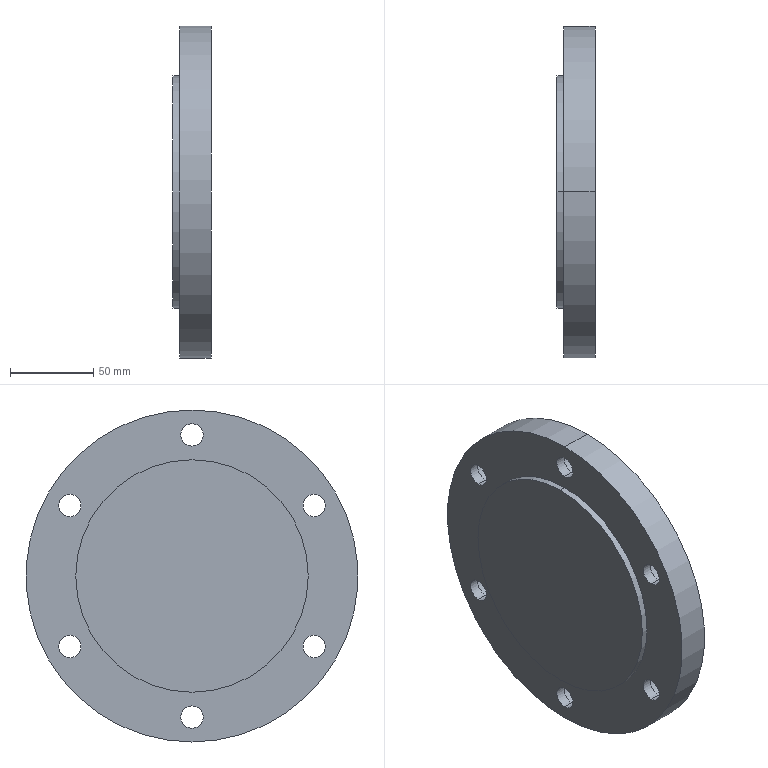Component | SolidWorks | JF21-80.1-30-1-SOLID1-1 | 1 solid | 37 faces | box 23 x 200 x 200 mm | volume 623674 mm3 | cylinder 28 | plane 9 | commonest cylinder face diameters 13.5 x12 22 x12 140 x2 200 x2
STEP:
#1=CARTESIAN_POINT('',(17.244,2.898,23.022));
#2=VERTEX_POINT('',#1);
#3=CARTESIAN_POINT('',(17.244,2.898,23.553));
#4=VERTEX_POINT('',#3);
#5=CARTESIAN_POINT('',(17.244,2.898,23.287));
#6=DIRECTION('',(-1.,0.,0.));
#7=DIRECTION('',(0.,0.,1.));
#8=AXIS2_PLACEMENT_3D('',#5,#6,#7);
#9=CIRCLE('',#8,0.2657);
#10=EDGE_CURVE('',#2,#4,#9,.T.);
#11=ORIENTED_EDGE('',*,*,#10,.T.);
#12=CARTESIAN_POINT('',(17.48,2.898,23.553));
#13=VERTEX_POINT('',#12);
#14=CARTESIAN_POINT('',(17.992,2.898,23.553));
#15=DIRECTION('',(-1.,0.,0.));
#16=VECTOR('',#15,39.37);
#17=LINE('',#14,#16);
#18=EDGE_CURVE('',#13,#4,#17,.T.);
#19=ORIENTED_EDGE('',*,*,#18,.F.);
#20=CARTESIAN_POINT('',(17.48,2.898,23.022));
#21=VERTEX_POINT('',#20);
#22=CARTESIAN_POINT('',(17.48,2.898,23.287));
#23=DIRECTION('',(1.,0.,0.));
#24=DIRECTION('',(0.,0.,-1.));
#25=AXIS2_PLACEMENT_3D('',#22,#23,#24);
#26=CIRCLE('',#25,0.2657);
#27=EDGE_CURVE('',#13,#21,#26,.T.);
#28=ORIENTED_EDGE('',*,*,#27,.T.);
#29=CARTESIAN_POINT('',(17.992,2.898,23.022));
#30=DIRECTION('',(-1.,0.,0.));
#31=VECTOR('',#30,39.37);
#32=LINE('',#29,#31);
#33=EDGE_CURVE('',#21,#2,#32,.T.);
#34=ORIENTED_EDGE('',*,*,#33,.T.);
#35=EDGE_LOOP('',(#11,#19,#28,#34));
#36=FACE_OUTER_BOUND('',#35,.T.);
#37=CARTESIAN_POINT('',(17.992,2.898,23.287));
#38=DIRECTION('',(1.,0.,0.));
#39=DIRECTION('',(0.,0.,1.));
#40=AXIS2_PLACEMENT_3D('',#37,#38,#39);
#41=CYLINDRICAL_SURFACE('',#40,0.2657);
#42=ADVANCED_FACE('',(#36),#41,.F.);
#43=CARTESIAN_POINT('',(17.48,2.898,23.72));
#44=VERTEX_POINT('',#43);
#45=CARTESIAN_POINT('',(17.48,2.898,22.854));
#46=VERTEX_POINT('',#45);
#47=CARTESIAN_POINT('',(17.48,2.898,23.287));
#48=DIRECTION('',(1.,0.,0.));
#49=DIRECTION('',(0.,0.,-1.));
#50=AXIS2_PLACEMENT_3D('',#47,#48,#49);
#51=CIRCLE('',#50,0.4331);
#52=EDGE_CURVE('',#44,#46,#51,.T.);
#53=ORIENTED_EDGE('',*,*,#52,.F.);
#54=CARTESIAN_POINT('',(17.992,2.898,23.72));
#55=VERTEX_POINT('',#54);
#56=CARTESIAN_POINT('',(17.992,2.898,23.72));
#57=DIRECTION('',(-1.,0.,0.));
#58=VECTOR('',#57,39.37);
#59=LINE('',#56,#58);
#60=EDGE_CURVE('',#55,#44,#59,.T.);
#61=ORIENTED_EDGE('',*,*,#60,.F.);
#62=CARTESIAN_POINT('',(17.992,2.898,22.854));
#63=VERTEX_POINT('',#62);
#64=CARTESIAN_POINT('',(17.992,2.898,23.287));
#65=DIRECTION('',(1.,0.,0.));
#66=DIRECTION('',(0.,0.,-1.));
#67=AXIS2_PLACEMENT_3D('',#64,#65,#66);
#68=CIRCLE('',#67,0.4331);
#69=EDGE_CURVE('',#55,#63,#68,.T.);
#70=ORIENTED_EDGE('',*,*,#69,.T.);
#71=CARTESIAN_POINT('',(17.992,2.898,22.854));
#72=DIRECTION('',(-1.,0.,0.));
#73=VECTOR('',#72,39.37);
#74=LINE('',#71,#73);
#75=EDGE_CURVE('',#63,#46,#74,.T.);
#76=ORIENTED_EDGE('',*,*,#75,.T.);
#77=EDGE_LOOP('',(#53,#61,#70,#76));
#78=FACE_OUTER_BOUND('',#77,.T.);
#79=CARTESIAN_POINT('',(17.992,2.898,23.287));
#80=DIRECTION('',(1.,0.,0.));
#81=DIRECTION('',(0.,0.,1.));
#82=AXIS2_PLACEMENT_3D('',#79,#80,#81);
#83=CYLINDRICAL_SURFACE('',#82,0.4331);
#84=ADVANCED_FACE('',(#78),#83,.F.);
#85=CARTESIAN_POINT('',(17.244,2.898,19.675));
#86=VERTEX_POINT('',#85);
#87=CARTESIAN_POINT('',(17.244,2.898,20.207));
#88=VERTEX_POINT('',#87);
#89=CARTESIAN_POINT('',(17.244,2.898,19.941));
#90=DIRECTION('',(-1.,0.,0.));
#91=DIRECTION('',(0.,0.,1.));
#92=AXIS2_PLACEMENT_3D('',#89,#90,#91);
#93=CIRCLE('',#92,0.2657);
#94=EDGE_CURVE('',#86,#88,#93,.T.);
#95=ORIENTED_EDGE('',*,*,#94,.T.);
#96=CARTESIAN_POINT('',(17.48,2.898,20.207));
#97=VERTEX_POINT('',#96);
#98=CARTESIAN_POINT('',(17.992,2.898,20.207));
#99=DIRECTION('',(-1.,0.,0.));
#100=VECTOR('',#99,39.37);
#101=LINE('',#98,#100);
#102=EDGE_CURVE('',#97,#88,#101,.T.);
#103=ORIENTED_EDGE('',*,*,#102,.F.);
#104=CARTESIAN_POINT('',(17.48,2.898,19.675));
#105=VERTEX_POINT('',#104);
#106=CARTESIAN_POINT('',(17.48,2.898,19.941));
#107=DIRECTION('',(1.,0.,0.));
#108=DIRECTION('',(0.,0.,-1.));
#109=AXIS2_PLACEMENT_3D('',#106,#107,#108);
#110=CIRCLE('',#109,0.2657);
#111=EDGE_CURVE('',#97,#105,#110,.T.);
#112=ORIENTED_EDGE('',*,*,#111,.T.);
#113=CARTESIAN_POINT('',(17.992,2.898,19.675));
#114=DIRECTION('',(-1.,0.,0.));
#115=VECTOR('',#114,39.37);
#116=LINE('',#113,#115);
#117=EDGE_CURVE('',#105,#86,#116,.T.);
#118=ORIENTED_EDGE('',*,*,#117,.T.);
#119=EDGE_LOOP('',(#95,#103,#112,#118));
#120=FACE_OUTER_BOUND('',#119,.T.);
#121=CARTESIAN_POINT('',(17.992,2.898,19.941));
#122=DIRECTION('',(1.,0.,0.));
#123=DIRECTION('',(0.,0.,1.));
#124=AXIS2_PLACEMENT_3D('',#121,#122,#123);
#125=CYLINDRICAL_SURFACE('',#124,0.2657);
#126=ADVANCED_FACE('',(#120),#125,.F.);
#127=CARTESIAN_POINT('',(17.48,2.898,20.374));
#128=VERTEX_POINT('',#127);
#129=CARTESIAN_POINT('',(17.48,2.898,19.508));
#130=VERTEX_POINT('',#129);
#131=CARTESIAN_POINT('',(17.48,2.898,19.941));
#132=DIRECTION('',(1.,0.,0.));
#133=DIRECTION('',(0.,0.,-1.));
#134=AXIS2_PLACEMENT_3D('',#131,#132,#133);
#135=CIRCLE('',#134,0.4331);
#136=EDGE_CURVE('',#128,#130,#135,.T.);
#137=ORIENTED_EDGE('',*,*,#136,.F.);
#138=CARTESIAN_POINT('',(17.992,2.898,20.374));
#139=VERTEX_POINT('',#138);
#140=CARTESIAN_POINT('',(17.992,2.898,20.374));
#141=DIRECTION('',(-1.,0.,0.));
#142=VECTOR('',#141,39.37);
#143=LINE('',#140,#142);
#144=EDGE_CURVE('',#139,#128,#143,.T.);
#145=ORIENTED_EDGE('',*,*,#144,.F.);
#146=CARTESIAN_POINT('',(17.992,2.898,19.508));
#147=VERTEX_POINT('',#146);
#148=CARTESIAN_POINT('',(17.992,2.898,19.941));
#149=DIRECTION('',(1.,0.,0.));
#150=DIRECTION('',(0.,0.,-1.));
#151=AXIS2_PLACEMENT_3D('',#148,#149,#150);
#152=CIRCLE('',#151,0.4331);
#153=EDGE_CURVE('',#139,#147,#152,.T.);
#154=ORIENTED_EDGE('',*,*,#153,.T.);
#155=CARTESIAN_POINT('',(17.992,2.898,19.508));
#156=DIRECTION('',(-1.,0.,0.));
#157=VECTOR('',#156,39.37);
#158=LINE('',#155,#157);
#159=EDGE_CURVE('',#147,#130,#158,.T.);
#160=ORIENTED_EDGE('',*,*,#159,.T.);
#161=EDGE_LOOP('',(#137,#145,#154,#160));
#162=FACE_OUTER_BOUND('',#161,.T.);
#163=CARTESIAN_POINT('',(17.992,2.898,19.941));
#164=DIRECTION('',(1.,0.,0.));
#165=DIRECTION('',(0.,0.,1.));
#166=AXIS2_PLACEMENT_3D('',#163,#164,#165);
#167=CYLINDRICAL_SURFACE('',#166,0.4331);
#168=ADVANCED_FACE('',(#162),#167,.F.);
#169=CARTESIAN_POINT('',(17.244,-0.,18.002));
#170=VERTEX_POINT('',#169);
#171=CARTESIAN_POINT('',(17.244,-0.,18.533));
#172=VERTEX_POINT('',#171);
#173=CARTESIAN_POINT('',(17.244,-0.,18.268));
#174=DIRECTION('',(-1.,0.,0.));
#175=DIRECTION('',(0.,0.,1.));
#176=AXIS2_PLACEMENT_3D('',#173,#174,#175);
#177=CIRCLE('',#176,0.2657);
#178=EDGE_CURVE('',#170,#172,#177,.T.);
#179=ORIENTED_EDGE('',*,*,#178,.T.);
#180=CARTESIAN_POINT('',(17.48,-0.,18.533));
#181=VERTEX_POINT('',#180);
#182=CARTESIAN_POINT('',(17.992,-0.,18.533));
#183=DIRECTION('',(-1.,0.,0.));
#184=VECTOR('',#183,39.37);
#185=LINE('',#182,#184);
#186=EDGE_CURVE('',#181,#172,#185,.T.);
#187=ORIENTED_EDGE('',*,*,#186,.F.);
#188=CARTESIAN_POINT('',(17.48,-0.,18.002));
#189=VERTEX_POINT('',#188);
#190=CARTESIAN_POINT('',(17.48,-0.,18.268));
#191=DIRECTION('',(1.,0.,0.));
#192=DIRECTION('',(0.,0.,-1.));
#193=AXIS2_PLACEMENT_3D('',#190,#191,#192);
#194=CIRCLE('',#193,0.2657);
#195=EDGE_CURVE('',#181,#189,#194,.T.);
#196=ORIENTED_EDGE('',*,*,#195,.T.);
#197=CARTESIAN_POINT('',(17.992,-0.,18.002));
#198=DIRECTION('',(-1.,0.,0.));
#199=VECTOR('',#198,39.37);
#200=LINE('',#197,#199);
#201=EDGE_CURVE('',#189,#170,#200,.T.);
#202=ORIENTED_EDGE('',*,*,#201,.T.);
#203=EDGE_LOOP('',(#179,#187,#196,#202));
#204=FACE_OUTER_BOUND('',#203,.T.);
#205=CARTESIAN_POINT('',(17.992,-0.,18.268));
#206=DIRECTION('',(1.,0.,0.));
#207=DIRECTION('',(0.,0.,1.));
#208=AXIS2_PLACEMENT_3D('',#205,#206,#207);
#209=CYLINDRICAL_SURFACE('',#208,0.2657);
#210=ADVANCED_FACE('',(#204),#209,.F.);
#211=CARTESIAN_POINT('',(17.48,-0.,18.701));
#212=VERTEX_POINT('',#211);
#213=CARTESIAN_POINT('',(17.48,-0.,17.835));
#214=VERTEX_POINT('',#213);
#215=CARTESIAN_POINT('',(17.48,-0.,18.268));
#216=DIRECTION('',(1.,0.,0.));
#217=DIRECTION('',(0.,0.,-1.));
#218=AXIS2_PLACEMENT_3D('',#215,#216,#217);
#219=CIRCLE('',#218,0.4331);
#220=EDGE_CURVE('',#212,#214,#219,.T.);
#221=ORIENTED_EDGE('',*,*,#220,.F.);
#222=CARTESIAN_POINT('',(17.992,-0.,18.701));
#223=VERTEX_POINT('',#222);
#224=CARTESIAN_POINT('',(17.992,-0.,18.701));
#225=DIRECTION('',(-1.,0.,0.));
#226=VECTOR('',#225,39.37);
#227=LINE('',#224,#226);
#228=EDGE_CURVE('',#223,#212,#227,.T.);
#229=ORIENTED_EDGE('',*,*,#228,.F.);
#230=CARTESIAN_POINT('',(17.992,-0.,17.835));
#231=VERTEX_POINT('',#230);
#232=CARTESIAN_POINT('',(17.992,-0.,18.268));
#233=DIRECTION('',(1.,0.,0.));
#234=DIRECTION('',(0.,0.,-1.));
#235=AXIS2_PLACEMENT_3D('',#232,#233,#234);
#236=CIRCLE('',#235,0.4331);
#237=EDGE_CURVE('',#223,#231,#236,.T.);
#238=ORIENTED_EDGE('',*,*,#237,.T.);
#239=CARTESIAN_POINT('',(17.992,-0.,17.835));
#240=DIRECTION('',(-1.,0.,0.));
#241=VECTOR('',#240,39.37);
#242=LINE('',#239,#241);
#243=EDGE_CURVE('',#231,#214,#242,.T.);
#244=ORIENTED_EDGE('',*,*,#243,.T.);
#245=EDGE_LOOP('',(#221,#229,#238,#244));
#246=FACE_OUTER_BOUND('',#245,.T.);
#247=CARTESIAN_POINT('',(17.992,-0.,18.268));
#248=DIRECTION('',(1.,0.,0.));
#249=DIRECTION('',(0.,0.,1.));
#250=AXIS2_PLACEMENT_3D('',#247,#248,#249);
#251=CYLINDRICAL_SURFACE('',#250,0.4331);
#252=ADVANCED_FACE('',(#246),#251,.F.);
#253=CARTESIAN_POINT('',(17.244,-2.898,19.675));
#254=VERTEX_POINT('',#253);
#255=CARTESIAN_POINT('',(17.244,-2.898,20.207));
#256=VERTEX_POINT('',#255);
#257=CARTESIAN_POINT('',(17.244,-2.898,19.941));
#258=DIRECTION('',(-1.,0.,0.));
#259=DIRECTION('',(0.,0.,1.));
#260=AXIS2_PLACEMENT_3D('',#257,#258,#259);
#261=CIRCLE('',#260,0.2657);
#262=EDGE_CURVE('',#254,#256,#261,.T.);
#263=ORIENTED_EDGE('',*,*,#262,.T.);
#264=CARTESIAN_POINT('',(17.48,-2.898,20.207));
#265=VERTEX_POINT('',#264);
#266=CARTESIAN_POINT('',(17.992,-2.898,20.207));
#267=DIRECTION('',(-1.,0.,0.));
#268=VECTOR('',#267,39.37);
#269=LINE('',#266,#268);
#270=EDGE_CURVE('',#265,#256,#269,.T.);
#271=ORIENTED_EDGE('',*,*,#270,.F.);
#272=CARTESIAN_POINT('',(17.48,-2.898,19.675));
#273=VERTEX_POINT('',#272);
#274=CARTESIAN_POINT('',(17.48,-2.898,19.941));
#275=DIRECTION('',(1.,0.,0.));
#276=DIRECTION('',(0.,0.,-1.));
#277=AXIS2_PLACEMENT_3D('',#274,#275,#276);
#278=CIRCLE('',#277,0.2657);
#279=EDGE_CURVE('',#265,#273,#278,.T.);
#280=ORIENTED_EDGE('',*,*,#279,.T.);
#281=CARTESIAN_POINT('',(17.992,-2.898,19.675));
#282=DIRECTION('',(-1.,0.,0.));
#283=VECTOR('',#282,39.37);
#284=LINE('',#281,#283);
#285=EDGE_CURVE('',#273,#254,#284,.T.);
#286=ORIENTED_EDGE('',*,*,#285,.T.);
#287=EDGE_LOOP('',(#263,#271,#280,#286));
#288=FACE_OUTER_BOUND('',#287,.T.);
#289=CARTESIAN_POINT('',(17.992,-2.898,19.941));
#290=DIRECTION('',(1.,0.,0.));
#291=DIRECTION('',(0.,0.,1.));
#292=AXIS2_PLACEMENT_3D('',#289,#290,#291);
#293=CYLINDRICAL_SURFACE('',#292,0.2657);
#294=ADVANCED_FACE('',(#288),#293,.F.);
#295=CARTESIAN_POINT('',(17.48,-2.898,20.374));
#296=VERTEX_POINT('',#295);
#297=CARTESIAN_POINT('',(17.48,-2.898,19.508));
#298=VERTEX_POINT('',#297);
#299=CARTESIAN_POINT('',(17.48,-2.898,19.941));
#300=DIRECTION('',(1.,0.,0.));
#301=DIRECTION('',(0.,0.,-1.));
#302=AXIS2_PLACEMENT_3D('',#299,#300,#301);
#303=CIRCLE('',#302,0.4331);
#304=EDGE_CURVE('',#296,#298,#303,.T.);
#305=ORIENTED_EDGE('',*,*,#304,.F.);
#306=CARTESIAN_POINT('',(17.992,-2.898,20.374));
#307=VERTEX_POINT('',#306);
#308=CARTESIAN_POINT('',(17.992,-2.898,20.374));
#309=DIRECTION('',(-1.,0.,0.));
#310=VECTOR('',#309,39.37);
#311=LINE('',#308,#310);
#312=EDGE_CURVE('',#307,#296,#311,.T.);
#313=ORIENTED_EDGE('',*,*,#312,.F.);
#314=CARTESIAN_POINT('',(17.992,-2.898,19.508));
#315=VERTEX_POINT('',#314);
#316=CARTESIAN_POINT('',(17.992,-2.898,19.941));
#317=DIRECTION('',(1.,0.,0.));
#318=DIRECTION('',(0.,0.,-1.));
#319=AXIS2_PLACEMENT_3D('',#316,#317,#318);
#320=CIRCLE('',#319,0.4331);
#321=EDGE_CURVE('',#307,#315,#320,.T.);
#322=ORIENTED_EDGE('',*,*,#321,.T.);
#323=CARTESIAN_POINT('',(17.992,-2.898,19.508));
#324=DIRECTION('',(-1.,0.,0.));
#325=VECTOR('',#324,39.37);
#326=LINE('',#323,#325);
#327=EDGE_CURVE('',#315,#298,#326,.T.);
#328=ORIENTED_EDGE('',*,*,#327,.T.);
#329=EDGE_LOOP('',(#305,#313,#322,#328));
#330=FACE_OUTER_BOUND('',#329,.T.);
#331=CARTESIAN_POINT('',(17.992,-2.898,19.941));
#332=DIRECTION('',(1.,0.,0.));
#333=DIRECTION('',(0.,0.,1.));
#334=AXIS2_PLACEMENT_3D('',#331,#332,#333);
#335=CYLINDRICAL_SURFACE('',#334,0.4331);
#336=ADVANCED_FACE('',(#330),#335,.F.);
#337=CARTESIAN_POINT('',(17.244,-2.898,23.022));
#338=VERTEX_POINT('',#337);
#339=CARTESIAN_POINT('',(17.244,-2.898,23.553));
#340=VERTEX_POINT('',#339);
#341=CARTESIAN_POINT('',(17.244,-2.898,23.287));
#342=DIRECTION('',(-1.,0.,0.));
#343=DIRECTION('',(0.,0.,1.));
#344=AXIS2_PLACEMENT_3D('',#341,#342,#343);
#345=CIRCLE('',#344,0.2657);
#346=EDGE_CURVE('',#338,#340,#345,.T.);
#347=ORIENTED_EDGE('',*,*,#346,.T.);
#348=CARTESIAN_POINT('',(17.48,-2.898,23.553));
#349=VERTEX_POINT('',#348);
#350=CARTESIAN_POINT('',(17.992,-2.898,23.553));
#351=DIRECTION('',(-1.,0.,0.));
#352=VECTOR('',#351,39.37);
#353=LINE('',#350,#352);
#354=EDGE_CURVE('',#349,#340,#353,.T.);
#355=ORIENTED_EDGE('',*,*,#354,.F.);
#356=CARTESIAN_POINT('',(17.48,-2.898,23.022));
#357=VERTEX_POINT('',#356);
#358=CARTESIAN_POINT('',(17.48,-2.898,23.287));
#359=DIRECTION('',(1.,0.,0.));
#360=DIRECTION('',(0.,0.,-1.));
#361=AXIS2_PLACEMENT_3D('',#358,#359,#360);
#362=CIRCLE('',#361,0.2657);
#363=EDGE_CURVE('',#349,#357,#362,.T.);
#364=ORIENTED_EDGE('',*,*,#363,.T.);
#365=CARTESIAN_POINT('',(17.992,-2.898,23.022));
#366=DIRECTION('',(-1.,0.,0.));
#367=VECTOR('',#366,39.37);
#368=LINE('',#365,#367);
#369=EDGE_CURVE('',#357,#338,#368,.T.);
#370=ORIENTED_EDGE('',*,*,#369,.T.);
#371=EDGE_LOOP('',(#347,#355,#364,#370));
#372=FACE_OUTER_BOUND('',#371,.T.);
#373=CARTESIAN_POINT('',(17.992,-2.898,23.287));
#374=DIRECTION('',(1.,0.,0.));
#375=DIRECTION('',(0.,0.,1.));
#376=AXIS2_PLACEMENT_3D('',#373,#374,#375);
#377=CYLINDRICAL_SURFACE('',#376,0.2657);
#378=ADVANCED_FACE('',(#372),#377,.F.);
#379=CARTESIAN_POINT('',(17.48,-2.898,23.72));
#380=VERTEX_POINT('',#379);
#381=CARTESIAN_POINT('',(17.48,-2.898,22.854));
#382=VERTEX_POINT('',#381);
#383=CARTESIAN_POINT('',(17.48,-2.898,23.287));
#384=DIRECTION('',(1.,0.,0.));
#385=DIRECTION('',(0.,0.,-1.));
#386=AXIS2_PLACEMENT_3D('',#383,#384,#385);
#387=CIRCLE('',#386,0.4331);
#388=EDGE_CURVE('',#380,#382,#387,.T.);
#389=ORIENTED_EDGE('',*,*,#388,.F.);
#390=CARTESIAN_POINT('',(17.992,-2.898,23.72));
#391=VERTEX_POINT('',#390);
#392=CARTESIAN_POINT('',(17.992,-2.898,23.72));
#393=DIRECTION('',(-1.,0.,0.));
#394=VECTOR('',#393,39.37);
#395=LINE('',#392,#394);
#396=EDGE_CURVE('',#391,#380,#395,.T.);
#397=ORIENTED_EDGE('',*,*,#396,.F.);
#398=CARTESIAN_POINT('',(17.992,-2.898,22.854));
#399=VERTEX_POINT('',#398);
#400=CARTESIAN_POINT('',(17.992,-2.898,23.287));
#401=DIRECTION('',(1.,0.,0.));
#402=DIRECTION('',(0.,0.,-1.));
#403=AXIS2_PLACEMENT_3D('',#400,#401,#402);
#404=CIRCLE('',#403,0.4331);
#405=EDGE_CURVE('',#391,#399,#404,.T.);
#406=ORIENTED_EDGE('',*,*,#405,.T.);
#407=CARTESIAN_POINT('',(17.992,-2.898,22.854));
#408=DIRECTION('',(-1.,0.,0.));
#409=VECTOR('',#408,39.37);
#410=LINE('',#407,#409);
#411=EDGE_CURVE('',#399,#382,#410,.T.);
#412=ORIENTED_EDGE('',*,*,#411,.T.);
#413=EDGE_LOOP('',(#389,#397,#406,#412));
#414=FACE_OUTER_BOUND('',#413,.T.);
#415=CARTESIAN_POINT('',(17.992,-2.898,23.287));
#416=DIRECTION('',(1.,0.,0.));
#417=DIRECTION('',(0.,0.,1.));
#418=AXIS2_PLACEMENT_3D('',#415,#416,#417);
#419=CYLINDRICAL_SURFACE('',#418,0.4331);
#420=ADVANCED_FACE('',(#414),#419,.F.);
#421=CARTESIAN_POINT('',(17.244,-0.,24.695));
#422=VERTEX_POINT('',#421);
#423=CARTESIAN_POINT('',(17.244,-0.,25.226));
#424=VERTEX_POINT('',#423);
#425=CARTESIAN_POINT('',(17.244,-0.,24.961));
#426=DIRECTION('',(-1.,0.,0.));
#427=DIRECTION('',(0.,0.,1.));
#428=AXIS2_PLACEMENT_3D('',#425,#426,#427);
#429=CIRCLE('',#428,0.2657);
#430=EDGE_CURVE('',#422,#424,#429,.T.);
#431=ORIENTED_EDGE('',*,*,#430,.T.);
#432=CARTESIAN_POINT('',(17.48,-0.,25.226));
#433=VERTEX_POINT('',#432);
#434=CARTESIAN_POINT('',(17.992,-0.,25.226));
#435=DIRECTION('',(-1.,0.,0.));
#436=VECTOR('',#435,39.37);
#437=LINE('',#434,#436);
#438=EDGE_CURVE('',#433,#424,#437,.T.);
#439=ORIENTED_EDGE('',*,*,#438,.F.);
#440=CARTESIAN_POINT('',(17.48,-0.,24.695));
#441=VERTEX_POINT('',#440);
#442=CARTESIAN_POINT('',(17.48,-0.,24.961));
#443=DIRECTION('',(1.,0.,0.));
#444=DIRECTION('',(0.,0.,-1.));
#445=AXIS2_PLACEMENT_3D('',#442,#443,#444);
#446=CIRCLE('',#445,0.2657);
#447=EDGE_CURVE('',#433,#441,#446,.T.);
#448=ORIENTED_EDGE('',*,*,#447,.T.);
#449=CARTESIAN_POINT('',(17.992,-0.,24.695));
#450=DIRECTION('',(-1.,0.,0.));
#451=VECTOR('',#450,39.37);
#452=LINE('',#449,#451);
#453=EDGE_CURVE('',#441,#422,#452,.T.);
#454=ORIENTED_EDGE('',*,*,#453,.T.);
#455=EDGE_LOOP('',(#431,#439,#448,#454));
#456=FACE_OUTER_BOUND('',#455,.T.);
#457=CARTESIAN_POINT('',(17.992,-0.,24.961));
#458=DIRECTION('',(1.,0.,0.));
#459=DIRECTION('',(0.,0.,1.));
#460=AXIS2_PLACEMENT_3D('',#457,#458,#459);
#461=CYLINDRICAL_SURFACE('',#460,0.2657);
#462=ADVANCED_FACE('',(#456),#461,.F.);
#463=CARTESIAN_POINT('',(17.48,-0.,25.394));
#464=VERTEX_POINT('',#463);
#465=CARTESIAN_POINT('',(17.48,-0.,24.528));
#466=VERTEX_POINT('',#465);
#467=CARTESIAN_POINT('',(17.48,-0.,24.961));
#468=DIRECTION('',(1.,0.,0.));
#469=DIRECTION('',(0.,0.,-1.));
#470=AXIS2_PLACEMENT_3D('',#467,#468,#469);
#471=CIRCLE('',#470,0.4331);
#472=EDGE_CURVE('',#464,#466,#471,.T.);
#473=ORIENTED_EDGE('',*,*,#472,.F.);
#474=CARTESIAN_POINT('',(17.992,-0.,25.394));
#475=VERTEX_POINT('',#474);
#476=CARTESIAN_POINT('',(17.992,-0.,25.394));
#477=DIRECTION('',(-1.,0.,0.));
#478=VECTOR('',#477,39.37);
#479=LINE('',#476,#478);
#480=EDGE_CURVE('',#475,#464,#479,.T.);
#481=ORIENTED_EDGE('',*,*,#480,.F.);
#482=CARTESIAN_POINT('',(17.992,-0.,24.528));
#483=VERTEX_POINT('',#482);
#484=CARTESIAN_POINT('',(17.992,-0.,24.961));
#485=DIRECTION('',(1.,0.,0.));
#486=DIRECTION('',(0.,0.,-1.));
#487=AXIS2_PLACEMENT_3D('',#484,#485,#486);
#488=CIRCLE('',#487,0.4331);
#489=EDGE_CURVE('',#475,#483,#488,.T.);
#490=ORIENTED_EDGE('',*,*,#489,.T.);
#491=CARTESIAN_POINT('',(17.992,-0.,24.528));
#492=DIRECTION('',(-1.,0.,0.));
#493=VECTOR('',#492,39.37);
#494=LINE('',#491,#493);
#495=EDGE_CURVE('',#483,#466,#494,.T.);
#496=ORIENTED_EDGE('',*,*,#495,.T.);
#497=EDGE_LOOP('',(#473,#481,#490,#496));
#498=FACE_OUTER_BOUND('',#497,.T.);
#499=CARTESIAN_POINT('',(17.992,-0.,24.961));
#500=DIRECTION('',(1.,0.,0.));
#501=DIRECTION('',(0.,0.,1.));
#502=AXIS2_PLACEMENT_3D('',#499,#500,#501);
#503=CYLINDRICAL_SURFACE('',#502,0.4331);
#504=ADVANCED_FACE('',(#498),#503,.F.);
#505=CARTESIAN_POINT('',(17.087,-0.,24.37));
#506=VERTEX_POINT('',#505);
#507=CARTESIAN_POINT('',(17.087,-0.,18.858));
#508=VERTEX_POINT('',#507);
#509=CARTESIAN_POINT('',(17.087,-0.,21.614));
#510=DIRECTION('',(-1.,0.,0.));
#511=DIRECTION('',(0.,0.,1.));
#512=AXIS2_PLACEMENT_3D('',#509,#510,#511);
#513=CIRCLE('',#512,2.756);
#514=EDGE_CURVE('',#506,#508,#513,.T.);
#515=ORIENTED_EDGE('',*,*,#514,.F.);
#516=CARTESIAN_POINT('',(17.244,-0.,24.37));
#517=VERTEX_POINT('',#516);
#518=CARTESIAN_POINT('',(17.087,-0.,24.37));
#519=DIRECTION('',(-1.,0.,0.));
#520=VECTOR('',#519,39.37);
#521=LINE('',#518,#520);
#522=EDGE_CURVE('',#517,#506,#521,.T.);
#523=ORIENTED_EDGE('',*,*,#522,.F.);
#524=CARTESIAN_POINT('',(17.244,-0.,18.858));
#525=VERTEX_POINT('',#524);
#526=CARTESIAN_POINT('',(17.244,-0.,21.614));
#527=DIRECTION('',(-1.,0.,0.));
#528=DIRECTION('',(0.,0.,1.));
#529=AXIS2_PLACEMENT_3D('',#526,#527,#528);
#530=CIRCLE('',#529,2.756);
#531=EDGE_CURVE('',#517,#525,#530,.T.);
#532=ORIENTED_EDGE('',*,*,#531,.T.);
#533=CARTESIAN_POINT('',(17.087,-0.,18.858));
#534=DIRECTION('',(-1.,0.,0.));
#535=VECTOR('',#534,39.37);
#536=LINE('',#533,#535);
#537=EDGE_CURVE('',#525,#508,#536,.T.);
#538=ORIENTED_EDGE('',*,*,#537,.T.);
#539=EDGE_LOOP('',(#515,#523,#532,#538));
#540=FACE_OUTER_BOUND('',#539,.T.);
#541=CARTESIAN_POINT('',(17.087,-0.,21.614));
#542=DIRECTION('',(1.,0.,0.));
#543=DIRECTION('',(0.,0.,1.));
#544=AXIS2_PLACEMENT_3D('',#541,#542,#543);
#545=CYLINDRICAL_SURFACE('',#544,2.756);
#546=ADVANCED_FACE('',(#540),#545,.T.);
#547=CARTESIAN_POINT('',(17.244,-0.,25.551));
#548=VERTEX_POINT('',#547);
#549=CARTESIAN_POINT('',(17.244,-0.,17.677));
#550=VERTEX_POINT('',#549);
#551=CARTESIAN_POINT('',(17.244,-0.,21.614));
#552=DIRECTION('',(-1.,0.,0.));
#553=DIRECTION('',(0.,0.,1.));
#554=AXIS2_PLACEMENT_3D('',#551,#552,#553);
#555=CIRCLE('',#554,3.937);
#556=EDGE_CURVE('',#548,#550,#555,.T.);
#557=ORIENTED_EDGE('',*,*,#556,.F.);
#558=CARTESIAN_POINT('',(17.992,-0.,25.551));
#559=VERTEX_POINT('',#558);
#560=CARTESIAN_POINT('',(17.244,-0.,25.551));
#561=DIRECTION('',(-1.,0.,0.));
#562=VECTOR('',#561,39.37);
#563=LINE('',#560,#562);
#564=EDGE_CURVE('',#559,#548,#563,.T.);
#565=ORIENTED_EDGE('',*,*,#564,.F.);
#566=CARTESIAN_POINT('',(17.992,-0.,17.677));
#567=VERTEX_POINT('',#566);
#568=CARTESIAN_POINT('',(17.992,-0.,21.614));
#569=DIRECTION('',(-1.,0.,0.));
#570=DIRECTION('',(0.,0.,1.));
#571=AXIS2_PLACEMENT_3D('',#568,#569,#570);
#572=CIRCLE('',#571,3.937);
#573=EDGE_CURVE('',#559,#567,#572,.T.);
#574=ORIENTED_EDGE('',*,*,#573,.T.);
#575=CARTESIAN_POINT('',(17.244,-0.,17.677));
#576=DIRECTION('',(-1.,0.,0.));
#577=VECTOR('',#576,39.37);
#578=LINE('',#575,#577);
#579=EDGE_CURVE('',#567,#550,#578,.T.);
#580=ORIENTED_EDGE('',*,*,#579,.T.);
#581=EDGE_LOOP('',(#557,#565,#574,#580));
#582=FACE_OUTER_BOUND('',#581,.T.);
#583=CARTESIAN_POINT('',(17.244,-0.,21.614));
#584=DIRECTION('',(1.,0.,0.));
#585=DIRECTION('',(0.,0.,1.));
#586=AXIS2_PLACEMENT_3D('',#583,#584,#585);
#587=CYLINDRICAL_SURFACE('',#586,3.937);
#588=ADVANCED_FACE('',(#582),#587,.T.);
#589=ORIENTED_EDGE('',*,*,#10,.F.);
#590=CARTESIAN_POINT('',(17.244,2.898,23.287));
#591=DIRECTION('',(-1.,0.,0.));
#592=DIRECTION('',(0.,0.,1.));
#593=AXIS2_PLACEMENT_3D('',#590,#591,#592);
#594=CIRCLE('',#593,0.2657);
#595=EDGE_CURVE('',#4,#2,#594,.T.);
#596=ORIENTED_EDGE('',*,*,#595,.F.);
#597=EDGE_LOOP('',(#589,#596));
#598=FACE_BOUND('',#597,.T.);
#599=ORIENTED_EDGE('',*,*,#94,.F.);
#600=CARTESIAN_POINT('',(17.244,2.898,19.941));
#601=DIRECTION('',(-1.,0.,0.));
#602=DIRECTION('',(0.,0.,1.));
#603=AXIS2_PLACEMENT_3D('',#600,#601,#602);
#604=CIRCLE('',#603,0.2657);
#605=EDGE_CURVE('',#88,#86,#604,.T.);
#606=ORIENTED_EDGE('',*,*,#605,.F.);
#607=EDGE_LOOP('',(#599,#606));
#608=FACE_BOUND('',#607,.T.);
#609=ORIENTED_EDGE('',*,*,#178,.F.);
#610=CARTESIAN_POINT('',(17.244,-0.,18.268));
#611=DIRECTION('',(-1.,0.,0.));
#612=DIRECTION('',(0.,0.,1.));
#613=AXIS2_PLACEMENT_3D('',#610,#611,#612);
#614=CIRCLE('',#613,0.2657);
#615=EDGE_CURVE('',#172,#170,#614,.T.);
#616=ORIENTED_EDGE('',*,*,#615,.F.);
#617=EDGE_LOOP('',(#609,#616));
#618=FACE_BOUND('',#617,.T.);
#619=ORIENTED_EDGE('',*,*,#262,.F.);
#620=CARTESIAN_POINT('',(17.244,-2.898,19.941));
#621=DIRECTION('',(-1.,0.,0.));
#622=DIRECTION('',(0.,0.,1.));
#623=AXIS2_PLACEMENT_3D('',#620,#621,#622);
#624=CIRCLE('',#623,0.2657);
#625=EDGE_CURVE('',#256,#254,#624,.T.);
#626=ORIENTED_EDGE('',*,*,#625,.F.);
#627=EDGE_LOOP('',(#619,#626));
#628=FACE_BOUND('',#627,.T.);
#629=ORIENTED_EDGE('',*,*,#346,.F.);
#630=CARTESIAN_POINT('',(17.244,-2.898,23.287));
#631=DIRECTION('',(-1.,0.,0.));
#632=DIRECTION('',(0.,0.,1.));
#633=AXIS2_PLACEMENT_3D('',#630,#631,#632);
#634=CIRCLE('',#633,0.2657);
#635=EDGE_CURVE('',#340,#338,#634,.T.);
#636=ORIENTED_EDGE('',*,*,#635,.F.);
#637=EDGE_LOOP('',(#629,#636));
#638=FACE_BOUND('',#637,.T.);
#639=ORIENTED_EDGE('',*,*,#430,.F.);
#640=CARTESIAN_POINT('',(17.244,-0.,24.961));
#641=DIRECTION('',(-1.,0.,0.));
#642=DIRECTION('',(0.,0.,1.));
#643=AXIS2_PLACEMENT_3D('',#640,#641,#642);
#644=CIRCLE('',#643,0.2657);
#645=EDGE_CURVE('',#424,#422,#644,.T.);
#646=ORIENTED_EDGE('',*,*,#645,.F.);
#647=EDGE_LOOP('',(#639,#646));
#648=FACE_BOUND('',#647,.T.);
#649=CARTESIAN_POINT('',(17.244,-0.,21.614));
#650=DIRECTION('',(-1.,0.,0.));
#651=DIRECTION('',(0.,0.,1.));
#652=AXIS2_PLACEMENT_3D('',#649,#650,#651);
#653=CIRCLE('',#652,3.937);
#654=EDGE_CURVE('',#550,#548,#653,.T.);
#655=ORIENTED_EDGE('',*,*,#654,.T.);
#656=ORIENTED_EDGE('',*,*,#556,.T.);
#657=EDGE_LOOP('',(#655,#656));
#658=FACE_OUTER_BOUND('',#657,.T.);
#659=CARTESIAN_POINT('',(17.244,-0.,21.614));
#660=DIRECTION('',(-1.,0.,0.));
#661=DIRECTION('',(0.,0.,1.));
#662=AXIS2_PLACEMENT_3D('',#659,#660,#661);
#663=CIRCLE('',#662,2.756);
#664=EDGE_CURVE('',#525,#517,#663,.T.);
#665=ORIENTED_EDGE('',*,*,#664,.F.);
#666=ORIENTED_EDGE('',*,*,#531,.F.);
#667=EDGE_LOOP('',(#665,#666));
#668=FACE_BOUND('',#667,.T.);
#669=CARTESIAN_POINT('',(17.244,-0.,21.614));
#670=DIRECTION('',(-1.,0.,0.));
#671=DIRECTION('',(0.,0.,-1.));
#672=AXIS2_PLACEMENT_3D('',#669,#670,#671);
#673=PLANE('',#672);
#674=ADVANCED_FACE('',(#598,#608,#618,#628,#638,#648,#658,#668),#673,.T.);
#675=ORIENTED_EDGE('',*,*,#564,.T.);
#676=ORIENTED_EDGE('',*,*,#654,.F.);
#677=ORIENTED_EDGE('',*,*,#579,.F.);
#678=CARTESIAN_POINT('',(17.992,-0.,21.614));
#679=DIRECTION('',(-1.,0.,0.));
#680=DIRECTION('',(0.,0.,1.));
#681=AXIS2_PLACEMENT_3D('',#678,#679,#680);
#682=CIRCLE('',#681,3.937);
#683=EDGE_CURVE('',#567,#559,#682,.T.);
#684=ORIENTED_EDGE('',*,*,#683,.T.);
#685=EDGE_LOOP('',(#675,#676,#677,#684));
#686=FACE_OUTER_BOUND('',#685,.T.);
#687=CARTESIAN_POINT('',(17.244,-0.,21.614));
#688=DIRECTION('',(1.,0.,0.));
#689=DIRECTION('',(0.,0.,1.));
#690=AXIS2_PLACEMENT_3D('',#687,#688,#689);
#691=CYLINDRICAL_SURFACE('',#690,3.937);
#692=ADVANCED_FACE('',(#686),#691,.T.);
#693=CARTESIAN_POINT('',(17.992,2.898,23.287));
#694=DIRECTION('',(1.,0.,0.));
#695=DIRECTION('',(0.,0.,-1.));
#696=AXIS2_PLACEMENT_3D('',#693,#694,#695);
#697=CIRCLE('',#696,0.4331);
#698=EDGE_CURVE('',#63,#55,#697,.T.);
#699=ORIENTED_EDGE('',*,*,#698,.F.);
#700=ORIENTED_EDGE('',*,*,#69,.F.);
#701=EDGE_LOOP('',(#699,#700));
#702=FACE_BOUND('',#701,.T.);
#703=CARTESIAN_POINT('',(17.992,2.898,19.941));
#704=DIRECTION('',(1.,0.,0.));
#705=DIRECTION('',(0.,0.,-1.));
#706=AXIS2_PLACEMENT_3D('',#703,#704,#705);
#707=CIRCLE('',#706,0.4331);
#708=EDGE_CURVE('',#147,#139,#707,.T.);
#709=ORIENTED_EDGE('',*,*,#708,.F.);
#710=ORIENTED_EDGE('',*,*,#153,.F.);
#711=EDGE_LOOP('',(#709,#710));
#712=FACE_BOUND('',#711,.T.);
#713=CARTESIAN_POINT('',(17.992,-0.,18.268));
#714=DIRECTION('',(1.,0.,0.));
#715=DIRECTION('',(0.,0.,-1.));
#716=AXIS2_PLACEMENT_3D('',#713,#714,#715);
#717=CIRCLE('',#716,0.4331);
#718=EDGE_CURVE('',#231,#223,#717,.T.);
#719=ORIENTED_EDGE('',*,*,#718,.F.);
#720=ORIENTED_EDGE('',*,*,#237,.F.);
#721=EDGE_LOOP('',(#719,#720));
#722=FACE_BOUND('',#721,.T.);
#723=CARTESIAN_POINT('',(17.992,-2.898,19.941));
#724=DIRECTION('',(1.,0.,0.));
#725=DIRECTION('',(0.,0.,-1.));
#726=AXIS2_PLACEMENT_3D('',#723,#724,#725);
#727=CIRCLE('',#726,0.4331);
#728=EDGE_CURVE('',#315,#307,#727,.T.);
#729=ORIENTED_EDGE('',*,*,#728,.F.);
#730=ORIENTED_EDGE('',*,*,#321,.F.);
#731=EDGE_LOOP('',(#729,#730));
#732=FACE_BOUND('',#731,.T.);
#733=CARTESIAN_POINT('',(17.992,-2.898,23.287));
#734=DIRECTION('',(1.,0.,0.));
#735=DIRECTION('',(0.,0.,-1.));
#736=AXIS2_PLACEMENT_3D('',#733,#734,#735);
#737=CIRCLE('',#736,0.4331);
#738=EDGE_CURVE('',#399,#391,#737,.T.);
#739=ORIENTED_EDGE('',*,*,#738,.F.);
#740=ORIENTED_EDGE('',*,*,#405,.F.);
#741=EDGE_LOOP('',(#739,#740));
#742=FACE_BOUND('',#741,.T.);
#743=CARTESIAN_POINT('',(17.992,-0.,24.961));
#744=DIRECTION('',(1.,0.,0.));
#745=DIRECTION('',(0.,0.,-1.));
#746=AXIS2_PLACEMENT_3D('',#743,#744,#745);
#747=CIRCLE('',#746,0.4331);
#748=EDGE_CURVE('',#483,#475,#747,.T.);
#749=ORIENTED_EDGE('',*,*,#748,.F.);
#750=ORIENTED_EDGE('',*,*,#489,.F.);
#751=EDGE_LOOP('',(#749,#750));
#752=FACE_BOUND('',#751,.T.);
#753=ORIENTED_EDGE('',*,*,#683,.F.);
#754=ORIENTED_EDGE('',*,*,#573,.F.);
#755=EDGE_LOOP('',(#753,#754));
#756=FACE_OUTER_BOUND('',#755,.T.);
#757=CARTESIAN_POINT('',(17.992,-0.,21.614));
#758=DIRECTION('',(-1.,0.,0.));
#759=DIRECTION('',(0.,0.,-1.));
#760=AXIS2_PLACEMENT_3D('',#757,#758,#759);
#761=PLANE('',#760);
#762=ADVANCED_FACE('',(#702,#712,#722,#732,#742,#752,#756),#761,.F.);
#763=ORIENTED_EDGE('',*,*,#522,.T.);
#764=CARTESIAN_POINT('',(17.087,-0.,21.614));
#765=DIRECTION('',(-1.,0.,0.));
#766=DIRECTION('',(0.,0.,1.));
#767=AXIS2_PLACEMENT_3D('',#764,#765,#766);
#768=CIRCLE('',#767,2.756);
#769=EDGE_CURVE('',#508,#506,#768,.T.);
#770=ORIENTED_EDGE('',*,*,#769,.F.);
#771=ORIENTED_EDGE('',*,*,#537,.F.);
#772=ORIENTED_EDGE('',*,*,#664,.T.);
#773=EDGE_LOOP('',(#763,#770,#771,#772));
#774=FACE_OUTER_BOUND('',#773,.T.);
#775=CARTESIAN_POINT('',(17.087,-0.,21.614));
#776=DIRECTION('',(1.,0.,0.));
#777=DIRECTION('',(0.,0.,1.));
#778=AXIS2_PLACEMENT_3D('',#775,#776,#777);
#779=CYLINDRICAL_SURFACE('',#778,2.756);
#780=ADVANCED_FACE('',(#774),#779,.T.);
#781=ORIENTED_EDGE('',*,*,#769,.T.);
#782=ORIENTED_EDGE('',*,*,#514,.T.);
#783=EDGE_LOOP('',(#781,#782));
#784=FACE_OUTER_BOUND('',#783,.T.);
#785=CARTESIAN_POINT('',(17.087,-0.,21.614));
#786=DIRECTION('',(-1.,0.,0.));
#787=DIRECTION('',(0.,0.,-1.));
#788=AXIS2_PLACEMENT_3D('',#785,#786,#787);
#789=PLANE('',#788);
#790=ADVANCED_FACE('',(#784),#789,.T.);
#791=ORIENTED_EDGE('',*,*,#480,.T.);
#792=CARTESIAN_POINT('',(17.48,-0.,24.961));
#793=DIRECTION('',(1.,0.,0.));
#794=DIRECTION('',(0.,0.,-1.));
#795=AXIS2_PLACEMENT_3D('',#792,#793,#794);
#796=CIRCLE('',#795,0.4331);
#797=EDGE_CURVE('',#466,#464,#796,.T.);
#798=ORIENTED_EDGE('',*,*,#797,.F.);
#799=ORIENTED_EDGE('',*,*,#495,.F.);
#800=ORIENTED_EDGE('',*,*,#748,.T.);
#801=EDGE_LOOP('',(#791,#798,#799,#800));
#802=FACE_OUTER_BOUND('',#801,.T.);
#803=CARTESIAN_POINT('',(17.992,-0.,24.961));
#804=DIRECTION('',(1.,0.,0.));
#805=DIRECTION('',(0.,0.,1.));
#806=AXIS2_PLACEMENT_3D('',#803,#804,#805);
#807=CYLINDRICAL_SURFACE('',#806,0.4331);
#808=ADVANCED_FACE('',(#802),#807,.F.);
#809=CARTESIAN_POINT('',(17.48,-0.,24.961));
#810=DIRECTION('',(1.,0.,0.));
#811=DIRECTION('',(0.,0.,-1.));
#812=AXIS2_PLACEMENT_3D('',#809,#810,#811);
#813=CIRCLE('',#812,0.2657);
#814=EDGE_CURVE('',#441,#433,#813,.T.);
#815=ORIENTED_EDGE('',*,*,#814,.F.);
#816=ORIENTED_EDGE('',*,*,#447,.F.);
#817=EDGE_LOOP('',(#815,#816));
#818=FACE_BOUND('',#817,.T.);
#819=ORIENTED_EDGE('',*,*,#797,.T.);
#820=ORIENTED_EDGE('',*,*,#472,.T.);
#821=EDGE_LOOP('',(#819,#820));
#822=FACE_OUTER_BOUND('',#821,.T.);
#823=CARTESIAN_POINT('',(17.48,0.2657,24.961));
#824=DIRECTION('',(-1.,0.,0.));
#825=DIRECTION('',(0.,0.,-1.));
#826=AXIS2_PLACEMENT_3D('',#823,#824,#825);
#827=PLANE('',#826);
#828=ADVANCED_FACE('',(#818,#822),#827,.F.);
#829=ORIENTED_EDGE('',*,*,#438,.T.);
#830=ORIENTED_EDGE('',*,*,#645,.T.);
#831=ORIENTED_EDGE('',*,*,#453,.F.);
#832=ORIENTED_EDGE('',*,*,#814,.T.);
#833=EDGE_LOOP('',(#829,#830,#831,#832));
#834=FACE_OUTER_BOUND('',#833,.T.);
#835=CARTESIAN_POINT('',(17.992,-0.,24.961));
#836=DIRECTION('',(1.,0.,0.));
#837=DIRECTION('',(0.,0.,1.));
#838=AXIS2_PLACEMENT_3D('',#835,#836,#837);
#839=CYLINDRICAL_SURFACE('',#838,0.2657);
#840=ADVANCED_FACE('',(#834),#839,.F.);
#841=ORIENTED_EDGE('',*,*,#396,.T.);
#842=CARTESIAN_POINT('',(17.48,-2.898,23.287));
#843=DIRECTION('',(1.,0.,0.));
#844=DIRECTION('',(0.,0.,-1.));
#845=AXIS2_PLACEMENT_3D('',#842,#843,#844);
#846=CIRCLE('',#845,0.4331);
#847=EDGE_CURVE('',#382,#380,#846,.T.);
#848=ORIENTED_EDGE('',*,*,#847,.F.);
#849=ORIENTED_EDGE('',*,*,#411,.F.);
#850=ORIENTED_EDGE('',*,*,#738,.T.);
#851=EDGE_LOOP('',(#841,#848,#849,#850));
#852=FACE_OUTER_BOUND('',#851,.T.);
#853=CARTESIAN_POINT('',(17.992,-2.898,23.287));
#854=DIRECTION('',(1.,0.,0.));
#855=DIRECTION('',(0.,0.,1.));
#856=AXIS2_PLACEMENT_3D('',#853,#854,#855);
#857=CYLINDRICAL_SURFACE('',#856,0.4331);
#858=ADVANCED_FACE('',(#852),#857,.F.);
#859=CARTESIAN_POINT('',(17.48,-2.898,23.287));
#860=DIRECTION('',(1.,0.,0.));
#861=DIRECTION('',(0.,0.,-1.));
#862=AXIS2_PLACEMENT_3D('',#859,#860,#861);
#863=CIRCLE('',#862,0.2657);
#864=EDGE_CURVE('',#357,#349,#863,.T.);
#865=ORIENTED_EDGE('',*,*,#864,.F.);
#866=ORIENTED_EDGE('',*,*,#363,.F.);
#867=EDGE_LOOP('',(#865,#866));
#868=FACE_BOUND('',#867,.T.);
#869=ORIENTED_EDGE('',*,*,#847,.T.);
#870=ORIENTED_EDGE('',*,*,#388,.T.);
#871=EDGE_LOOP('',(#869,#870));
#872=FACE_OUTER_BOUND('',#871,.T.);
#873=CARTESIAN_POINT('',(17.48,-2.632,23.287));
#874=DIRECTION('',(-1.,0.,0.));
#875=DIRECTION('',(0.,0.,-1.));
#876=AXIS2_PLACEMENT_3D('',#873,#874,#875);
#877=PLANE('',#876);
#878=ADVANCED_FACE('',(#868,#872),#877,.F.);
#879=ORIENTED_EDGE('',*,*,#354,.T.);
#880=ORIENTED_EDGE('',*,*,#635,.T.);
#881=ORIENTED_EDGE('',*,*,#369,.F.);
#882=ORIENTED_EDGE('',*,*,#864,.T.);
#883=EDGE_LOOP('',(#879,#880,#881,#882));
#884=FACE_OUTER_BOUND('',#883,.T.);
#885=CARTESIAN_POINT('',(17.992,-2.898,23.287));
#886=DIRECTION('',(1.,0.,0.));
#887=DIRECTION('',(0.,0.,1.));
#888=AXIS2_PLACEMENT_3D('',#885,#886,#887);
#889=CYLINDRICAL_SURFACE('',#888,0.2657);
#890=ADVANCED_FACE('',(#884),#889,.F.);
#891=ORIENTED_EDGE('',*,*,#312,.T.);
#892=CARTESIAN_POINT('',(17.48,-2.898,19.941));
#893=DIRECTION('',(1.,0.,0.));
#894=DIRECTION('',(0.,0.,-1.));
#895=AXIS2_PLACEMENT_3D('',#892,#893,#894);
#896=CIRCLE('',#895,0.4331);
#897=EDGE_CURVE('',#298,#296,#896,.T.);
#898=ORIENTED_EDGE('',*,*,#897,.F.);
#899=ORIENTED_EDGE('',*,*,#327,.F.);
#900=ORIENTED_EDGE('',*,*,#728,.T.);
#901=EDGE_LOOP('',(#891,#898,#899,#900));
#902=FACE_OUTER_BOUND('',#901,.T.);
#903=CARTESIAN_POINT('',(17.992,-2.898,19.941));
#904=DIRECTION('',(1.,0.,0.));
#905=DIRECTION('',(0.,0.,1.));
#906=AXIS2_PLACEMENT_3D('',#903,#904,#905);
#907=CYLINDRICAL_SURFACE('',#906,0.4331);
#908=ADVANCED_FACE('',(#902),#907,.F.);
#909=CARTESIAN_POINT('',(17.48,-2.898,19.941));
#910=DIRECTION('',(1.,0.,0.));
#911=DIRECTION('',(0.,0.,-1.));
#912=AXIS2_PLACEMENT_3D('',#909,#910,#911);
#913=CIRCLE('',#912,0.2657);
#914=EDGE_CURVE('',#273,#265,#913,.T.);
#915=ORIENTED_EDGE('',*,*,#914,.F.);
#916=ORIENTED_EDGE('',*,*,#279,.F.);
#917=EDGE_LOOP('',(#915,#916));
#918=FACE_BOUND('',#917,.T.);
#919=ORIENTED_EDGE('',*,*,#897,.T.);
#920=ORIENTED_EDGE('',*,*,#304,.T.);
#921=EDGE_LOOP('',(#919,#920));
#922=FACE_OUTER_BOUND('',#921,.T.);
#923=CARTESIAN_POINT('',(17.48,-2.632,19.941));
#924=DIRECTION('',(-1.,0.,0.));
#925=DIRECTION('',(0.,0.,-1.));
#926=AXIS2_PLACEMENT_3D('',#923,#924,#925);
#927=PLANE('',#926);
#928=ADVANCED_FACE('',(#918,#922),#927,.F.);
#929=ORIENTED_EDGE('',*,*,#270,.T.);
#930=ORIENTED_EDGE('',*,*,#625,.T.);
#931=ORIENTED_EDGE('',*,*,#285,.F.);
#932=ORIENTED_EDGE('',*,*,#914,.T.);
#933=EDGE_LOOP('',(#929,#930,#931,#932));
#934=FACE_OUTER_BOUND('',#933,.T.);
#935=CARTESIAN_POINT('',(17.992,-2.898,19.941));
#936=DIRECTION('',(1.,0.,0.));
#937=DIRECTION('',(0.,0.,1.));
#938=AXIS2_PLACEMENT_3D('',#935,#936,#937);
#939=CYLINDRICAL_SURFACE('',#938,0.2657);
#940=ADVANCED_FACE('',(#934),#939,.F.);
#941=ORIENTED_EDGE('',*,*,#228,.T.);
#942=CARTESIAN_POINT('',(17.48,-0.,18.268));
#943=DIRECTION('',(1.,0.,0.));
#944=DIRECTION('',(0.,0.,-1.));
#945=AXIS2_PLACEMENT_3D('',#942,#943,#944);
#946=CIRCLE('',#945,0.4331);
#947=EDGE_CURVE('',#214,#212,#946,.T.);
#948=ORIENTED_EDGE('',*,*,#947,.F.);
#949=ORIENTED_EDGE('',*,*,#243,.F.);
#950=ORIENTED_EDGE('',*,*,#718,.T.);
#951=EDGE_LOOP('',(#941,#948,#949,#950));
#952=FACE_OUTER_BOUND('',#951,.T.);
#953=CARTESIAN_POINT('',(17.992,-0.,18.268));
#954=DIRECTION('',(1.,0.,0.));
#955=DIRECTION('',(0.,0.,1.));
#956=AXIS2_PLACEMENT_3D('',#953,#954,#955);
#957=CYLINDRICAL_SURFACE('',#956,0.4331);
#958=ADVANCED_FACE('',(#952),#957,.F.);
#959=CARTESIAN_POINT('',(17.48,-0.,18.268));
#960=DIRECTION('',(1.,0.,0.));
#961=DIRECTION('',(0.,0.,-1.));
#962=AXIS2_PLACEMENT_3D('',#959,#960,#961);
#963=CIRCLE('',#962,0.2657);
#964=EDGE_CURVE('',#189,#181,#963,.T.);
#965=ORIENTED_EDGE('',*,*,#964,.F.);
#966=ORIENTED_EDGE('',*,*,#195,.F.);
#967=EDGE_LOOP('',(#965,#966));
#968=FACE_BOUND('',#967,.T.);
#969=ORIENTED_EDGE('',*,*,#947,.T.);
#970=ORIENTED_EDGE('',*,*,#220,.T.);
#971=EDGE_LOOP('',(#969,#970));
#972=FACE_OUTER_BOUND('',#971,.T.);
#973=CARTESIAN_POINT('',(17.48,0.2657,18.268));
#974=DIRECTION('',(-1.,0.,0.));
#975=DIRECTION('',(0.,0.,-1.));
#976=AXIS2_PLACEMENT_3D('',#973,#974,#975);
#977=PLANE('',#976);
#978=ADVANCED_FACE('',(#968,#972),#977,.F.);
#979=ORIENTED_EDGE('',*,*,#186,.T.);
#980=ORIENTED_EDGE('',*,*,#615,.T.);
#981=ORIENTED_EDGE('',*,*,#201,.F.);
#982=ORIENTED_EDGE('',*,*,#964,.T.);
#983=EDGE_LOOP('',(#979,#980,#981,#982));
#984=FACE_OUTER_BOUND('',#983,.T.);
#985=CARTESIAN_POINT('',(17.992,-0.,18.268));
#986=DIRECTION('',(1.,0.,0.));
#987=DIRECTION('',(0.,0.,1.));
#988=AXIS2_PLACEMENT_3D('',#985,#986,#987);
#989=CYLINDRICAL_SURFACE('',#988,0.2657);
#990=ADVANCED_FACE('',(#984),#989,.F.);
#991=ORIENTED_EDGE('',*,*,#144,.T.);
#992=CARTESIAN_POINT('',(17.48,2.898,19.941));
#993=DIRECTION('',(1.,0.,0.));
#994=DIRECTION('',(0.,0.,-1.));
#995=AXIS2_PLACEMENT_3D('',#992,#993,#994);
#996=CIRCLE('',#995,0.4331);
#997=EDGE_CURVE('',#130,#128,#996,.T.);
#998=ORIENTED_EDGE('',*,*,#997,.F.);
#999=ORIENTED_EDGE('',*,*,#159,.F.);
#1000=ORIENTED_EDGE('',*,*,#708,.T.);
#1001=EDGE_LOOP('',(#991,#998,#999,#1000));
#1002=FACE_OUTER_BOUND('',#1001,.T.);
#1003=CARTESIAN_POINT('',(17.992,2.898,19.941));
#1004=DIRECTION('',(1.,0.,0.));
#1005=DIRECTION('',(0.,0.,1.));
#1006=AXIS2_PLACEMENT_3D('',#1003,#1004,#1005);
#1007=CYLINDRICAL_SURFACE('',#1006,0.4331);
#1008=ADVANCED_FACE('',(#1002),#1007,.F.);
#1009=CARTESIAN_POINT('',(17.48,2.898,19.941));
#1010=DIRECTION('',(1.,0.,0.));
#1011=DIRECTION('',(0.,0.,-1.));
#1012=AXIS2_PLACEMENT_3D('',#1009,#1010,#1011);
#1013=CIRCLE('',#1012,0.2657);
#1014=EDGE_CURVE('',#105,#97,#1013,.T.);
#1015=ORIENTED_EDGE('',*,*,#1014,.F.);
#1016=ORIENTED_EDGE('',*,*,#111,.F.);
#1017=EDGE_LOOP('',(#1015,#1016));
#1018=FACE_BOUND('',#1017,.T.);
#1019=ORIENTED_EDGE('',*,*,#997,.T.);
#1020=ORIENTED_EDGE('',*,*,#136,.T.);
#1021=EDGE_LOOP('',(#1019,#1020));
#1022=FACE_OUTER_BOUND('',#1021,.T.);
#1023=CARTESIAN_POINT('',(17.48,3.164,19.941));
#1024=DIRECTION('',(-1.,0.,0.));
#1025=DIRECTION('',(0.,0.,-1.));
#1026=AXIS2_PLACEMENT_3D('',#1023,#1024,#1025);
#1027=PLANE('',#1026);
#1028=ADVANCED_FACE('',(#1018,#1022),#1027,.F.);
#1029=ORIENTED_EDGE('',*,*,#102,.T.);
#1030=ORIENTED_EDGE('',*,*,#605,.T.);
#1031=ORIENTED_EDGE('',*,*,#117,.F.);
#1032=ORIENTED_EDGE('',*,*,#1014,.T.);
#1033=EDGE_LOOP('',(#1029,#1030,#1031,#1032));
#1034=FACE_OUTER_BOUND('',#1033,.T.);
#1035=CARTESIAN_POINT('',(17.992,2.898,19.941));
#1036=DIRECTION('',(1.,0.,0.));
#1037=DIRECTION('',(0.,0.,1.));
#1038=AXIS2_PLACEMENT_3D('',#1035,#1036,#1037);
#1039=CYLINDRICAL_SURFACE('',#1038,0.2657);
#1040=ADVANCED_FACE('',(#1034),#1039,.F.);
#1041=ORIENTED_EDGE('',*,*,#60,.T.);
#1042=CARTESIAN_POINT('',(17.48,2.898,23.287));
#1043=DIRECTION('',(1.,0.,0.));
#1044=DIRECTION('',(0.,0.,-1.));
#1045=AXIS2_PLACEMENT_3D('',#1042,#1043,#1044);
#1046=CIRCLE('',#1045,0.4331);
#1047=EDGE_CURVE('',#46,#44,#1046,.T.);
#1048=ORIENTED_EDGE('',*,*,#1047,.F.);
#1049=ORIENTED_EDGE('',*,*,#75,.F.);
#1050=ORIENTED_EDGE('',*,*,#698,.T.);
#1051=EDGE_LOOP('',(#1041,#1048,#1049,#1050));
#1052=FACE_OUTER_BOUND('',#1051,.T.);
#1053=CARTESIAN_POINT('',(17.992,2.898,23.287));
#1054=DIRECTION('',(1.,0.,0.));
#1055=DIRECTION('',(0.,0.,1.));
#1056=AXIS2_PLACEMENT_3D('',#1053,#1054,#1055);
#1057=CYLINDRICAL_SURFACE('',#1056,0.4331);
#1058=ADVANCED_FACE('',(#1052),#1057,.F.);
#1059=CARTESIAN_POINT('',(17.48,2.898,23.287));
#1060=DIRECTION('',(1.,0.,0.));
#1061=DIRECTION('',(0.,0.,-1.));
#1062=AXIS2_PLACEMENT_3D('',#1059,#1060,#1061);
#1063=CIRCLE('',#1062,0.2657);
#1064=EDGE_CURVE('',#21,#13,#1063,.T.);
#1065=ORIENTED_EDGE('',*,*,#1064,.F.);
#1066=ORIENTED_EDGE('',*,*,#27,.F.);
#1067=EDGE_LOOP('',(#1065,#1066));
#1068=FACE_BOUND('',#1067,.T.);
#1069=ORIENTED_EDGE('',*,*,#1047,.T.);
#1070=ORIENTED_EDGE('',*,*,#52,.T.);
#1071=EDGE_LOOP('',(#1069,#1070));
#1072=FACE_OUTER_BOUND('',#1071,.T.);
#1073=CARTESIAN_POINT('',(17.48,3.164,23.287));
#1074=DIRECTION('',(-1.,0.,0.));
#1075=DIRECTION('',(0.,0.,-1.));
#1076=AXIS2_PLACEMENT_3D('',#1073,#1074,#1075);
#1077=PLANE('',#1076);
#1078=ADVANCED_FACE('',(#1068,#1072),#1077,.F.);
#1079=ORIENTED_EDGE('',*,*,#18,.T.);
#1080=ORIENTED_EDGE('',*,*,#595,.T.);
#1081=ORIENTED_EDGE('',*,*,#33,.F.);
#1082=ORIENTED_EDGE('',*,*,#1064,.T.);
#1083=EDGE_LOOP('',(#1079,#1080,#1081,#1082));
#1084=FACE_OUTER_BOUND('',#1083,.T.);
#1085=CARTESIAN_POINT('',(17.992,2.898,23.287));
#1086=DIRECTION('',(1.,0.,0.));
#1087=DIRECTION('',(0.,0.,1.));
#1088=AXIS2_PLACEMENT_3D('',#1085,#1086,#1087);
#1089=CYLINDRICAL_SURFACE('',#1088,0.2657);
#1090=ADVANCED_FACE('',(#1084),#1089,.F.);
#1091=CLOSED_SHELL('',(#42,#84,#126,#168,#210,#252,#294,#336,#378,#420,#462,#504,#546,#588,#674,#692,#762,#780,#790,#808,#828,#840,#858,#878,#890,#908,#928,#940,#958,#978,#990,#1008,#1028,#1040,#1058,#1078,#1090));
#1092=MANIFOLD_SOLID_BREP('',#1091);
#1093=CARTESIAN_POINT('',(0.,0.,0.));
#1094=DIRECTION('',(0.,0.,1.));
#1095=DIRECTION('',(1.,0.,0.));
#1096=AXIS2_PLACEMENT_3D('',#1093,#1094,#1095);
#1097=(LENGTH_UNIT()NAMED_UNIT(*)SI_UNIT($,.METRE.));
#1098=LENGTH_MEASURE_WITH_UNIT(LENGTH_MEASURE(0.0254),#1097);
#1099=DIMENSIONAL_EXPONENTS(1.,0.,0.,0.,0.,0.,0.);
#1100=(CONVERSION_BASED_UNIT('',#1098)LENGTH_UNIT()NAMED_UNIT(#1099));
#1101=UNCERTAINTY_MEASURE_WITH_UNIT(LENGTH_MEASURE(0.00001),#1100,'','');
#1102=(NAMED_UNIT(*)PLANE_ANGLE_UNIT()SI_UNIT($,.RADIAN.));
#1103=(NAMED_UNIT(*)SI_UNIT($,.STERADIAN.)SOLID_ANGLE_UNIT());
#1104=(GEOMETRIC_REPRESENTATION_CONTEXT(3)GLOBAL_UNCERTAINTY_ASSIGNED_CONTEXT((#1101))GLOBAL_UNIT_ASSIGNED_CONTEXT((#1100,#1102,#1103))REPRESENTATION_CONTEXT('',''));
#1105=ADVANCED_BREP_SHAPE_REPRESENTATION('',(#1092,#1096),#1104);
#1106=COLOUR_RGB('',0.7922,0.8196,0.9333);
#1107=FILL_AREA_STYLE_COLOUR('',#1106);
#1108=FILL_AREA_STYLE('',(#1107));
#1109=SURFACE_STYLE_FILL_AREA(#1108);
#1110=SURFACE_SIDE_STYLE('',(#1109));
#1111=SURFACE_STYLE_USAGE(.BOTH.,#1110);
#1112=PRESENTATION_STYLE_ASSIGNMENT((#1111));
#1113=STYLED_ITEM('',(#1112),#1092);
#1114=(LENGTH_UNIT()NAMED_UNIT(*)SI_UNIT($,.METRE.));
#1115=LENGTH_MEASURE_WITH_UNIT(LENGTH_MEASURE(0.0254),#1114);
#1116=DIMENSIONAL_EXPONENTS(1.,0.,0.,0.,0.,0.,0.);
#1117=(CONVERSION_BASED_UNIT('',#1115)LENGTH_UNIT()NAMED_UNIT(#1116));
#1118=UNCERTAINTY_MEASURE_WITH_UNIT(LENGTH_MEASURE(0.00001),#1117,'','');
#1119=(NAMED_UNIT(*)PLANE_ANGLE_UNIT()SI_UNIT($,.RADIAN.));
#1120=(NAMED_UNIT(*)SI_UNIT($,.STERADIAN.)SOLID_ANGLE_UNIT());
#1121=(GEOMETRIC_REPRESENTATION_CONTEXT(3)GLOBAL_UNCERTAINTY_ASSIGNED_CONTEXT((#1118))GLOBAL_UNIT_ASSIGNED_CONTEXT((#1117,#1119,#1120))REPRESENTATION_CONTEXT('',''));
#1122=MECHANICAL_DESIGN_GEOMETRIC_PRESENTATION_REPRESENTATION('',(#1113),#1121);
#1123=PRESENTATION_LAYER_ASSIGNMENT('','',(#1113));